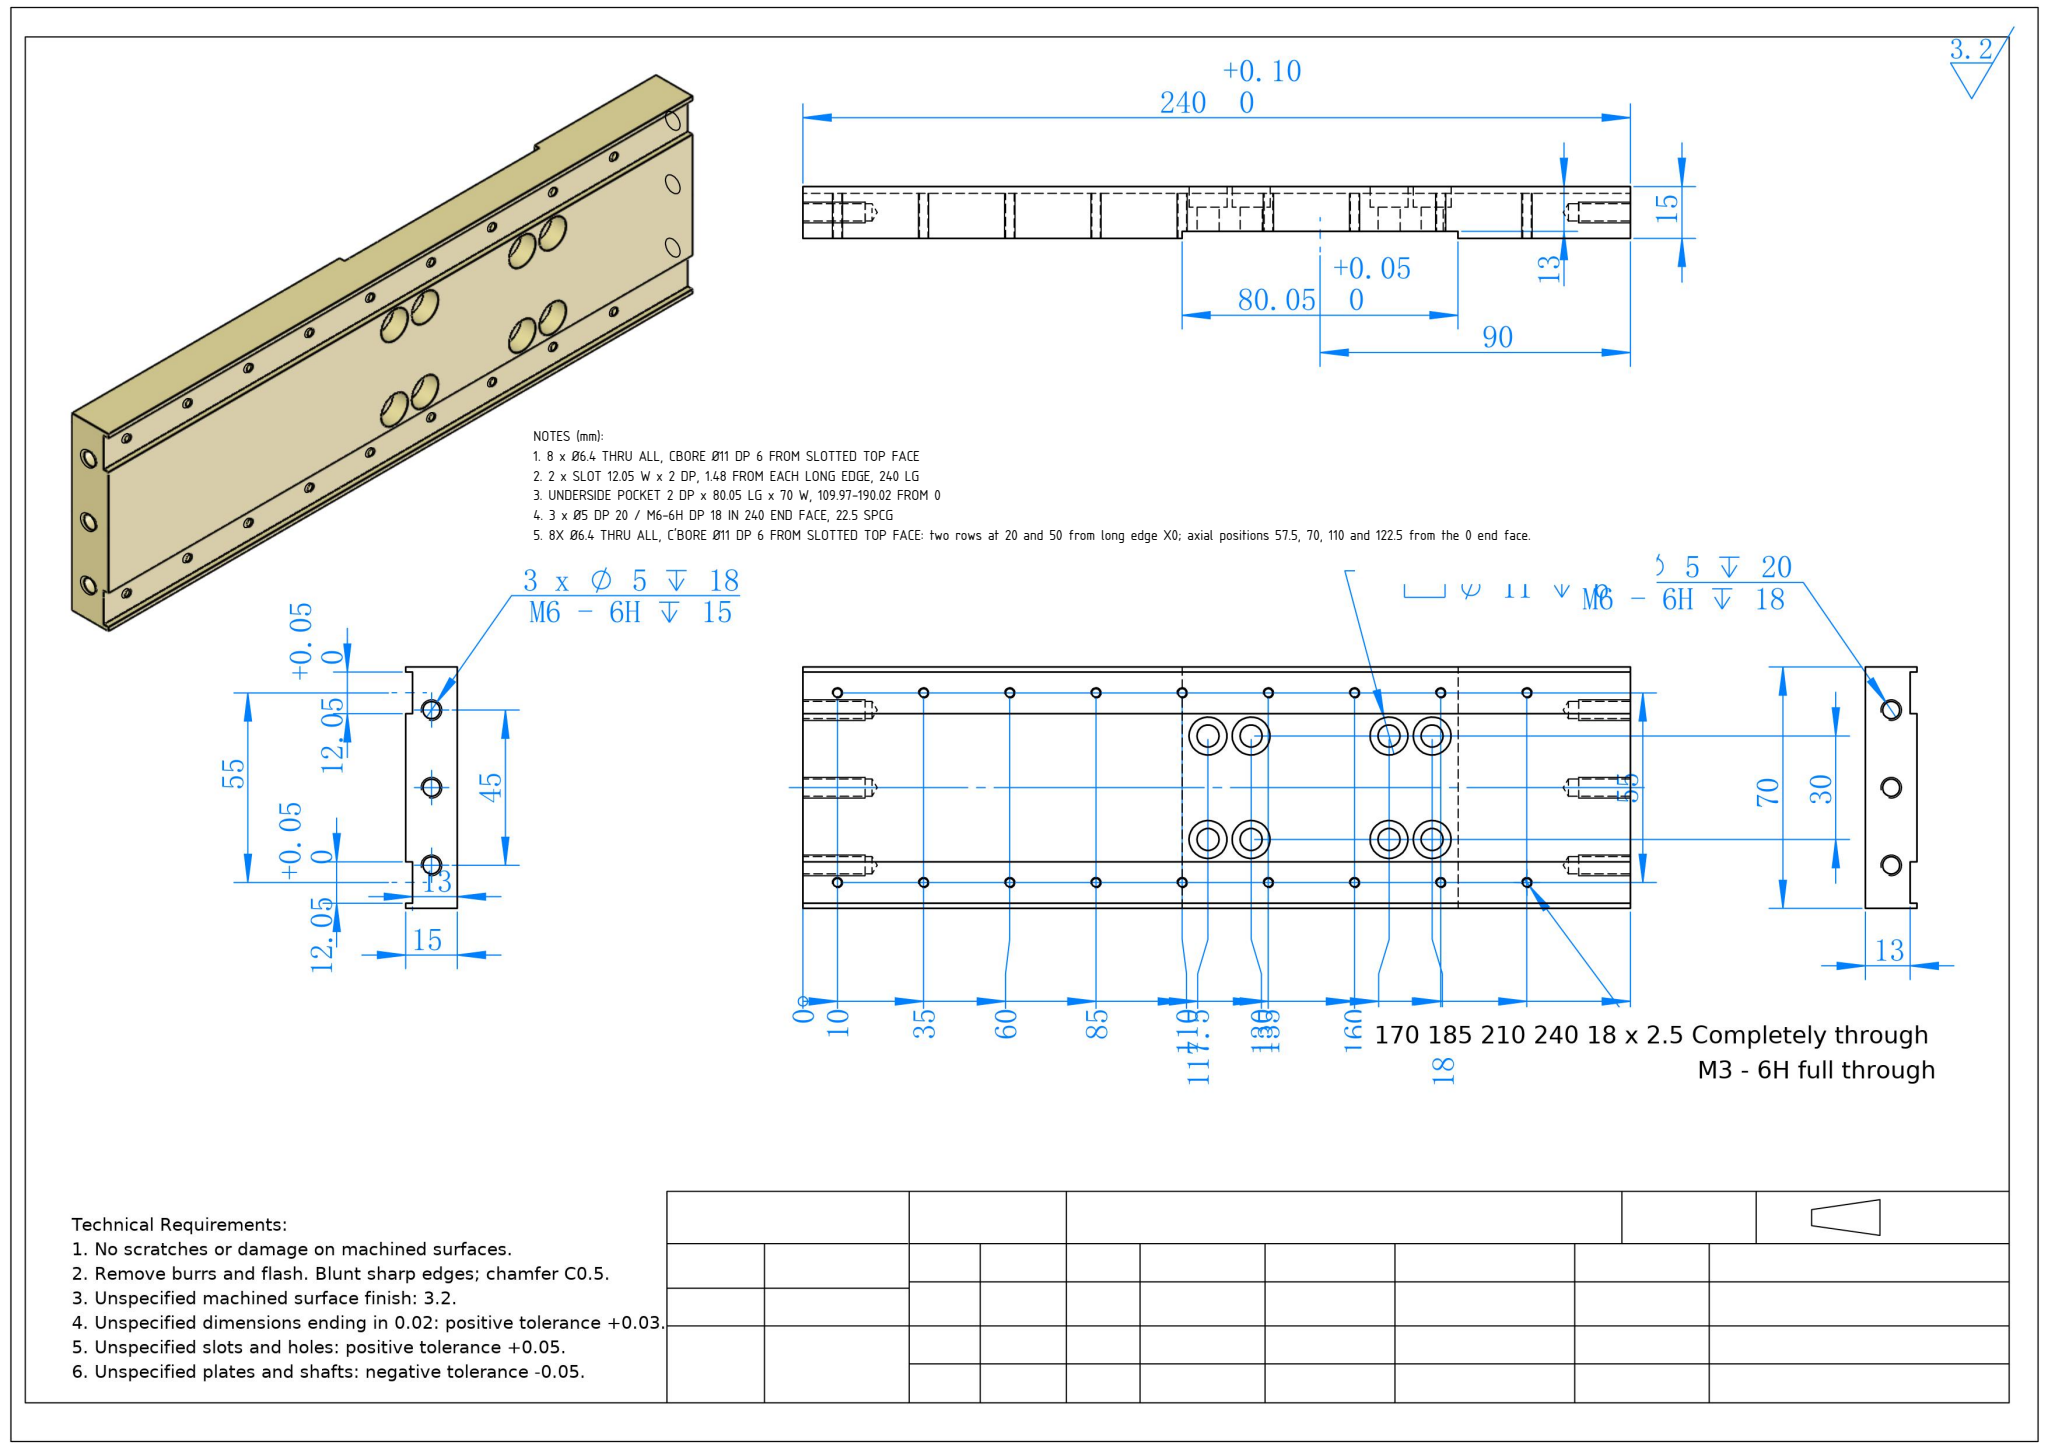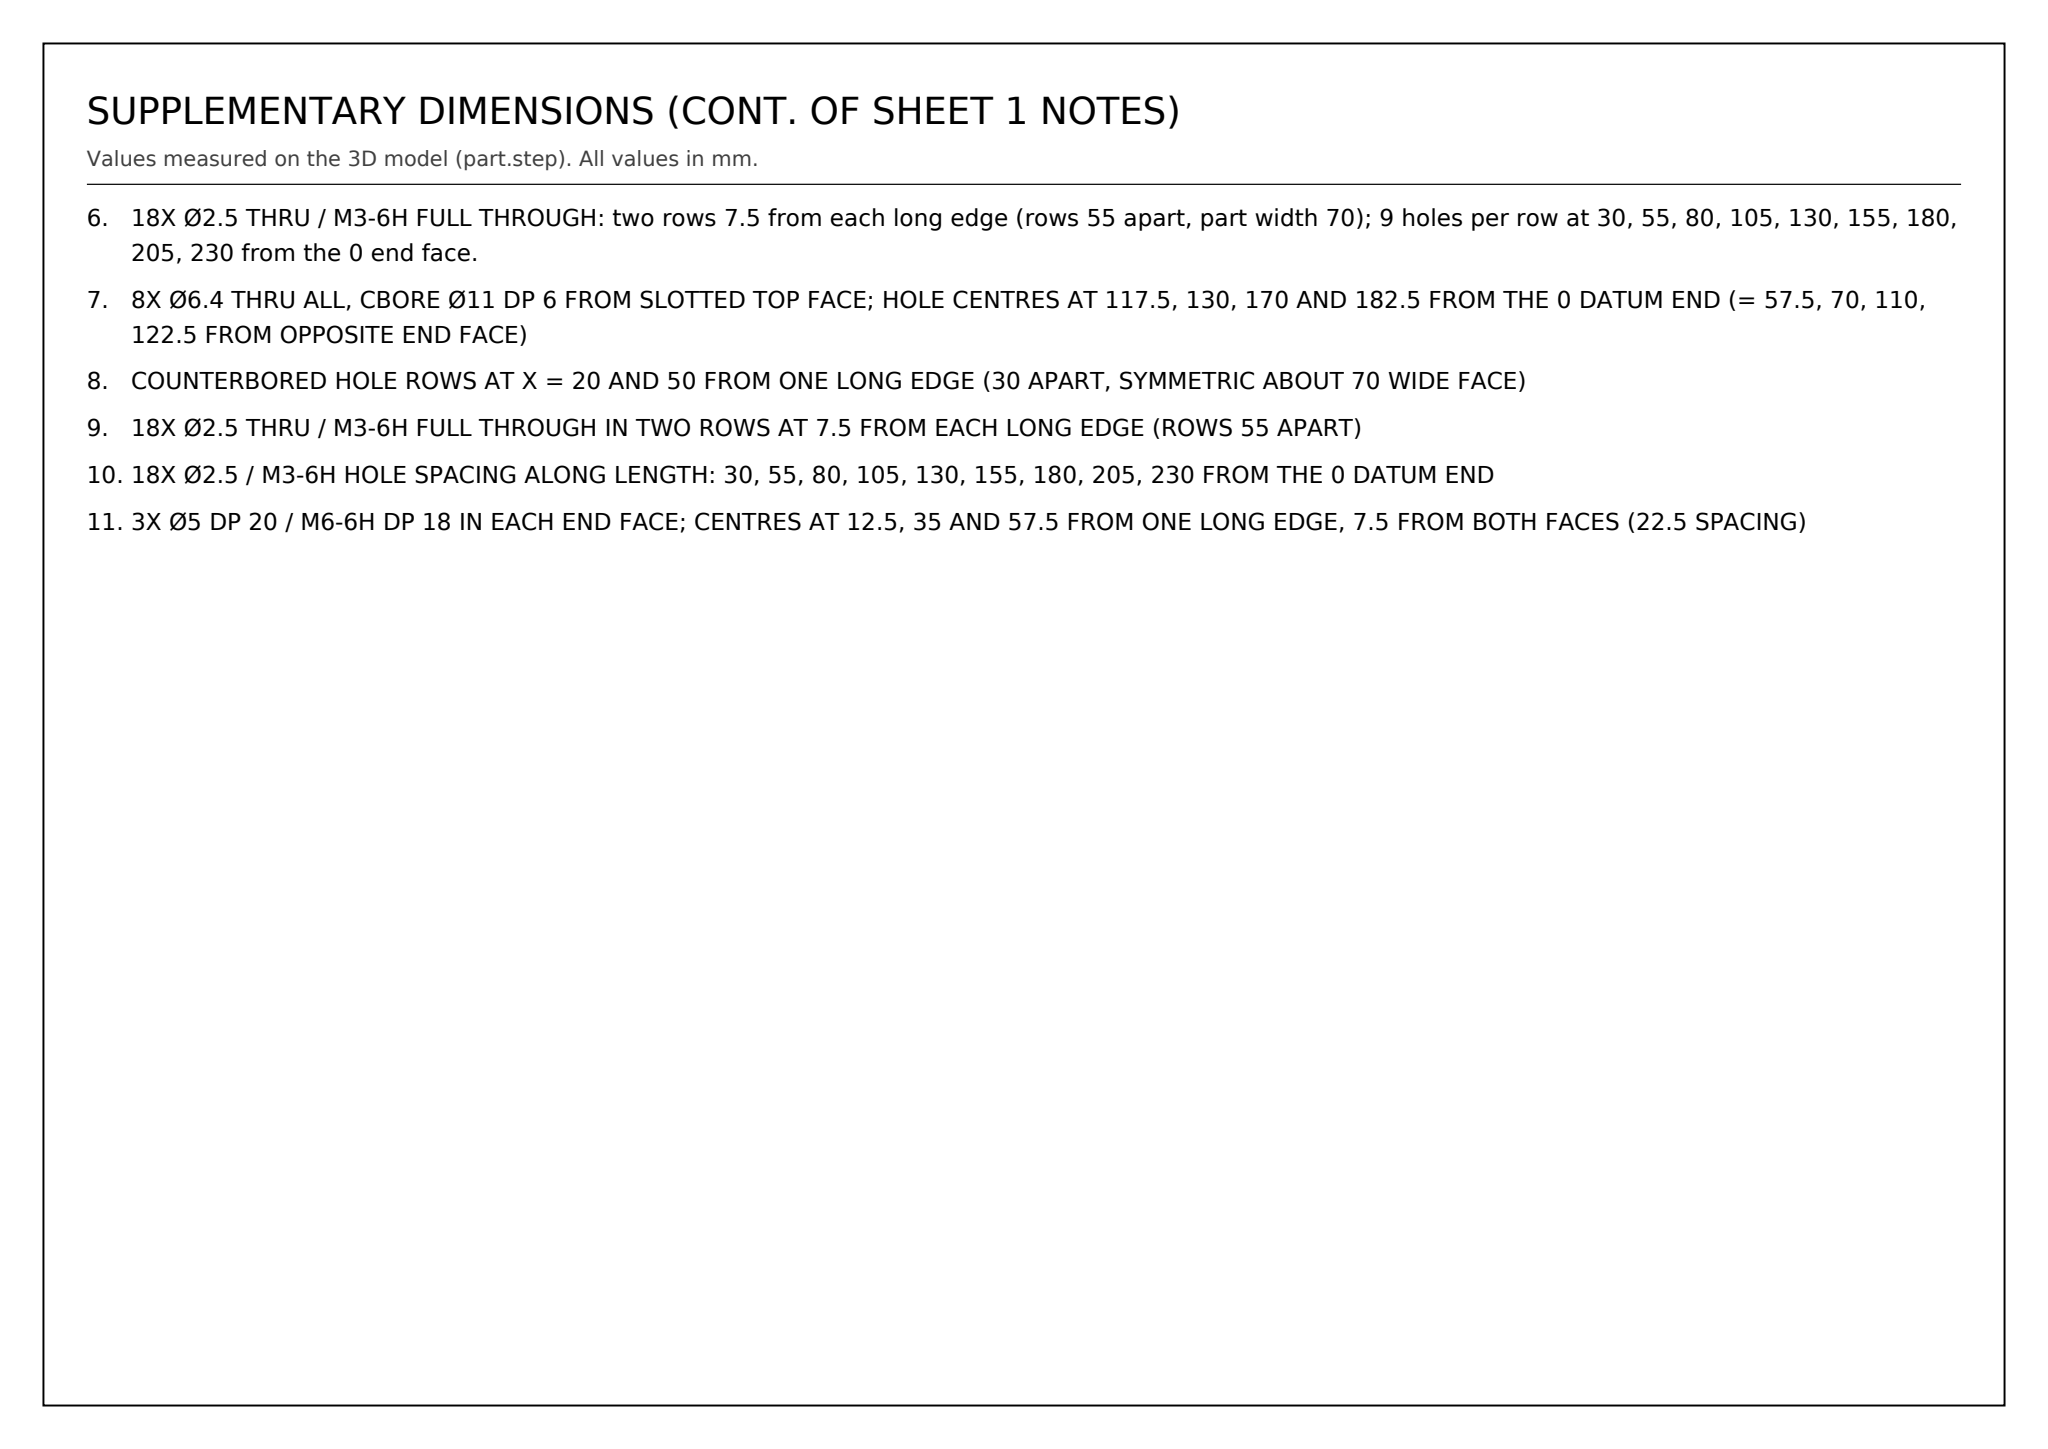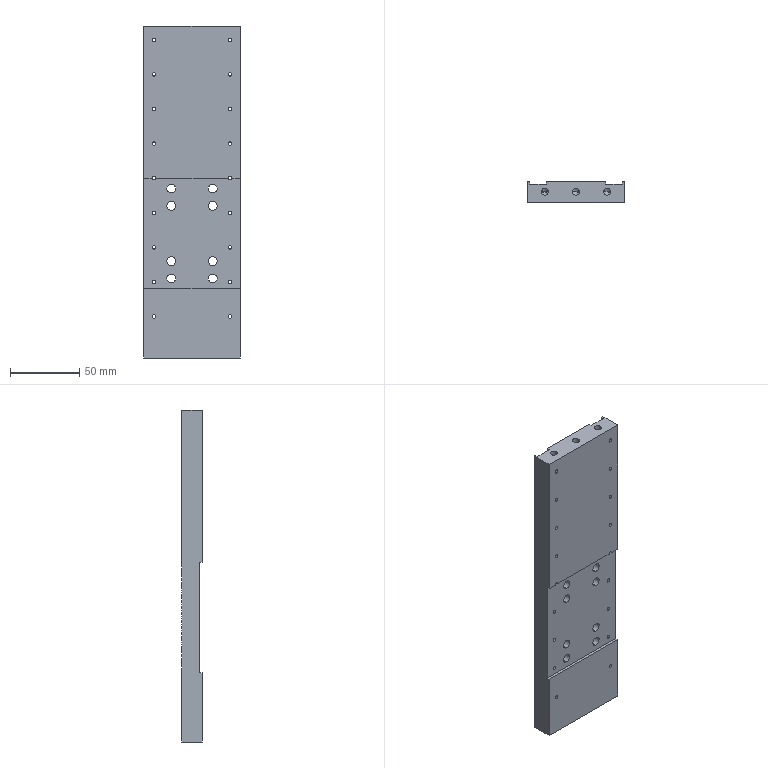Part | SolidWorks | mm | 1 solid | 120 faces | box 70 x 15 x 240 mm | volume 219485 mm3 | cylinder 80 | plane 28 | cone 12 | commonest cylinder face diameters 2.5 x36 11 x16 6.4 x16 5 x12
Drawing notes:
8 x Ø6.4 THRU ALL, CBORE Ø11 DP 6 FROM SLOTTED TOP FACE | from the solid: Ø6.4 y-holes L7 and Ø11 cbores L6 at x=20/50, z=57.5/70/110/122.5; cbore floors y=9.0, top face y=15.0
2 x SLOT 12.05 W x 2 DP, 1.48 FROM EACH LONG EDGE, 240 LG | from the solid: x planes 1.48/13.53 and 56.48/68.53 (12.05 wide), floors y=13.0 below top y=15.0, z=0 to 240
UNDERSIDE POCKET 2 DP x 80.05 LG x 70 W, 109.97-190.02 FROM 0 | from the solid: z planes 49.98 and 130.03 (80.05 apart) = dwg 190.02/109.97; floor y=2.0 from y=0 face, 13 thk left
3 x Ø5 DP 20 / M6-6H DP 18 IN 240 END FACE, 22.5 SPCG | from the solid: Ø5 z-axis holes L20 at x=12.5/35/57.5, y=7.5; 45 overall span, 22.5 pitch
8X Ø6.4 THRU ALL, C'BORE Ø11 DP 6 FROM SLOTTED TOP FACE: two rows at 20 and 50 from long edge X0; axial positions 57.5, 70, 110 and 122.5 from the 0 end face. | from the solid: cylinders dia 6.4 (len 7) and dia 11 (len 6), axis y, at x=20 and x=50, z=57.5, 70.0, 110.0, 122.5
18X Ø2.5 THRU / M3-6H FULL THROUGH: two rows 7.5 from each long edge (rows 55 apart, part width 70); 9 holes per row at 30, 55, 80, 105, 130, 155, 180, 205, 230 from the 0 end face. | from the solid: cylinders dia 2.5, axis y, at x=7.5 and x=62.5, z=30 through 230 in 25 steps (18 holes)
8X Ø6.4 THRU ALL, CBORE Ø11 DP 6 FROM SLOTTED TOP FACE; HOLE CENTRES AT 117.5, 130, 170 AND 182.5 FROM THE 0 DATUM END (= 57.5, 70, 110, 122.5 FROM OPPOSITE END FACE) | from the solid: cylinders dia 6.4 axis y at z=57.5/70/110/122.5 (len 7) and dia 11 axis y same z (len 6)
COUNTERBORED HOLE ROWS AT X = 20 AND 50 FROM ONE LONG EDGE (30 APART, SYMMETRIC ABOUT 70 WIDE FACE) | from the solid: cylinders dia 6.4 / dia 11 at x = 20.0 and 50.0
18X Ø2.5 THRU / M3-6H FULL THROUGH IN TWO ROWS AT 7.5 FROM EACH LONG EDGE (ROWS 55 APART) | from the solid: cylinders dia 2.5 axis y at x = 7.5 and 62.5 (bbox x = 70)
18X Ø2.5 / M3-6H HOLE SPACING ALONG LENGTH: 30, 55, 80, 105, 130, 155, 180, 205, 230 FROM THE 0 DATUM END | from the solid: cylinders dia 2.5 axis y at z = 30,55,80,105,130,155,180,205,230
3X Ø5 DP 20 / M6-6H DP 18 IN EACH END FACE; CENTRES AT 12.5, 35 AND 57.5 FROM ONE LONG EDGE, 7.5 FROM BOTH FACES (22.5 SPACING) | from the solid: cylinders dia 5 axis z at x=12.5/35.0/57.5, y=7.5, lengths 20 (drill) and 18 (thread), 2 instances each
build123d program:
from build123d import *

# Parameters (mm, degrees)
SKETCH1_W                                       = 70
SKETCH1_H                                       = 15
EXTRUDE1_DEPTH                                  = 120
SKETCH16_W                                      = 12.05
SKETCH16_H                                      = 240
CUT_EXTRUDE1_DEPTH                              = 2
SKETCH17_W                                      = 70
SKETCH17_H                                      = 80.05
CUT_EXTRUDE2_DEPTH                              = 2
M6_TAPPED_HOLE3_D                               = 5
M6_TAPPED_HOLE3_DEPTH                           = 18
M6_TAPPED_HOLE3_TIP                             = 1.502
M6_TAPPED_HOLE2_D                               = 5
M6_TAPPED_HOLE2_DEPTH                           = 20
M6_TAPPED_HOLE2_TIP                             = 1.502
M6_HEX_SOCKET_HEAD_CAP_SCREW_CBORE1_D           = 6.4
M6_HEX_SOCKET_HEAD_CAP_SCREW_CBORE1_CBORE_D     = 11
M6_HEX_SOCKET_HEAD_CAP_SCREW_CBORE1_CBORE_DEPTH = 6
M3_TAPPED_HOLE1_D                               = 2.5
LPATTERN1_COUNT                                 = 9
LPATTERN1_PITCH                                 = 25


with BuildPart() as part:
    # Sketch1 → Extrude1 (new, symmetric)
    with BuildSketch(Plane.XY):
        Rectangle(SKETCH1_W, SKETCH1_H)
    extrude(amount=EXTRUDE1_DEPTH, both=True)

    # Sketch16 → Cut-Extrude1 (cut)
    with BuildSketch(Plane(origin=(0, 7.5, 0), x_dir=(1, 0, 0), z_dir=(0, 1, 0))):
        with Locations((27.5, 0)):
            Rectangle(SKETCH16_W, SKETCH16_H)
        with Locations((-27.5, 0)):
            Rectangle(SKETCH16_W, SKETCH16_H)
    extrude(amount=-CUT_EXTRUDE1_DEPTH, mode=Mode.SUBTRACT)

    # Sketch17 → Cut-Extrude2 (cut)
    with BuildSketch(Plane(origin=(0, -7.5, 0), x_dir=(-1, 0, 0), z_dir=(0, -1, 0))):
        with Locations((0, 30)):
            Rectangle(SKETCH17_W, SKETCH17_H)
    extrude(amount=-CUT_EXTRUDE2_DEPTH, mode=Mode.SUBTRACT)

    # M6 Tapped Hole3
    with Locations(Plane(origin=(0, 0, -120), x_dir=(-1, 0, 0), z_dir=(0, 0, -1))):
        with Locations((-22.5, 0), (0, 0), (22.5, 0)):
            Hole(M6_TAPPED_HOLE3_D / 2, depth=M6_TAPPED_HOLE3_DEPTH)
            with Locations((0, 0, -(M6_TAPPED_HOLE3_DEPTH + M6_TAPPED_HOLE3_TIP / 2))):  # 118° drill point
                Cone(0, M6_TAPPED_HOLE3_D / 2, M6_TAPPED_HOLE3_TIP, mode=Mode.SUBTRACT)

    # M6 Tapped Hole2
    with Locations(Plane.XY.offset(120)):
        with Locations((-22.5, 0), (22.5, 0), (0, 0)):
            Hole(M6_TAPPED_HOLE2_D / 2, depth=M6_TAPPED_HOLE2_DEPTH)
            with Locations((0, 0, -(M6_TAPPED_HOLE2_DEPTH + M6_TAPPED_HOLE2_TIP / 2))):  # 118° drill point
                Cone(0, M6_TAPPED_HOLE2_D / 2, M6_TAPPED_HOLE2_TIP, mode=Mode.SUBTRACT)

    # M6 Hex Socket Head Cap Screw CBORE1 (through all)
    with Locations(Plane(origin=(0, 7.5, 0), x_dir=(1, 0, 0), z_dir=(0, 1, 0))):
        with Locations((15, 50), (-15, 50), (15, 10), (-15, 10), (-15, -2.5), (15, -2.5), (-15, 62.5), (15, 62.5)):
            CounterBoreHole(M6_HEX_SOCKET_HEAD_CAP_SCREW_CBORE1_D / 2, M6_HEX_SOCKET_HEAD_CAP_SCREW_CBORE1_CBORE_D / 2, M6_HEX_SOCKET_HEAD_CAP_SCREW_CBORE1_CBORE_DEPTH)

    # M3 Tapped Hole1 (through all)
    with Locations(Plane(origin=(0, 7.5, 0), x_dir=(-1, 0, 0), z_dir=(0, 1, 0))):
        with Locations((-27.5, -90), (27.5, -90)):
            m3_tapped_hole1 = Hole(M3_TAPPED_HOLE1_D / 2)

    # LPattern1: M3 Tapped Hole1 ×9
    with Locations(*[(0, 0, i * LPATTERN1_PITCH) for i in range(1, LPATTERN1_COUNT)]):
        add(m3_tapped_hole1, mode=Mode.SUBTRACT)


solid = part.part